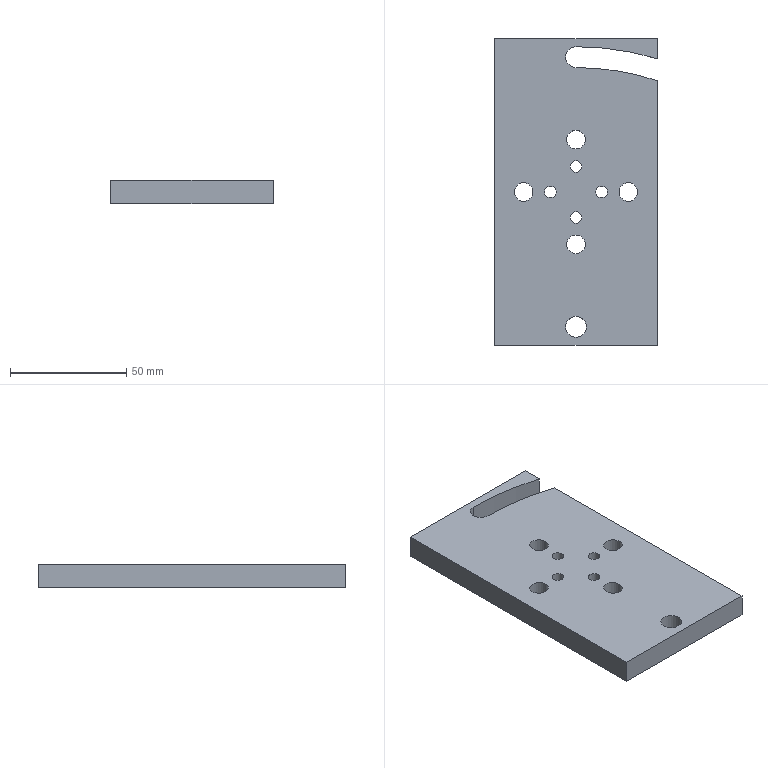Component | NX | DRILL_TEMPLATE | 1 solid | 19 faces | volume 85450 mm3 | cylinder 12 | plane 7 | commonest cylinder face diameters 8 x4 5 x4 9 x2 223 x1 241 x1